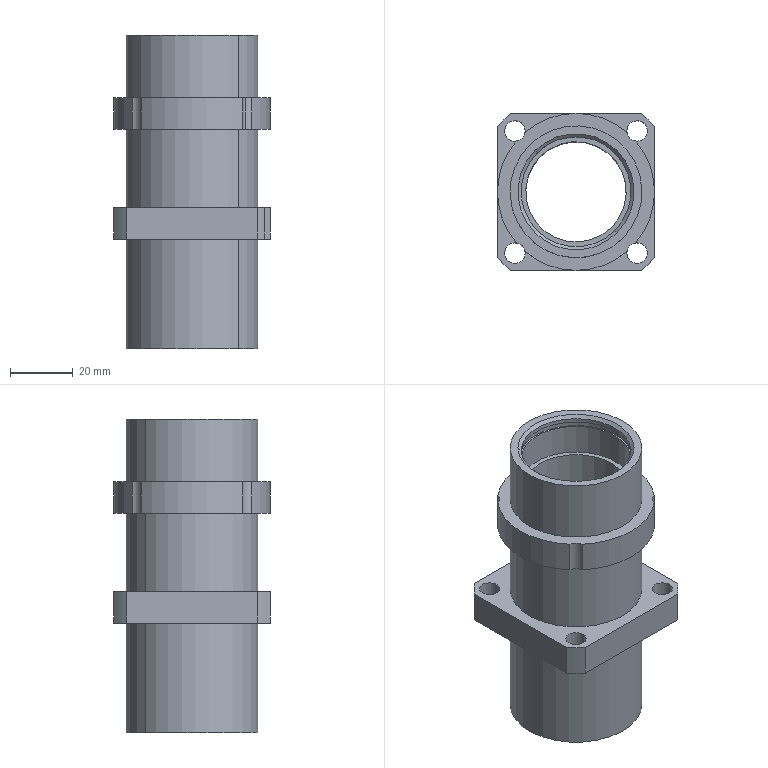Component | SolidWorks | DoubleFilmTransport-1_AxisSleeve-1 | 1 solid | 62 faces | volume 68579 mm3 | cylinder 42 | plane 16 | cone 4 | commonest cylinder face diameters 6.5 x13 35 x8 42 x6 65 x5 36 x4 50 x4 32 x2